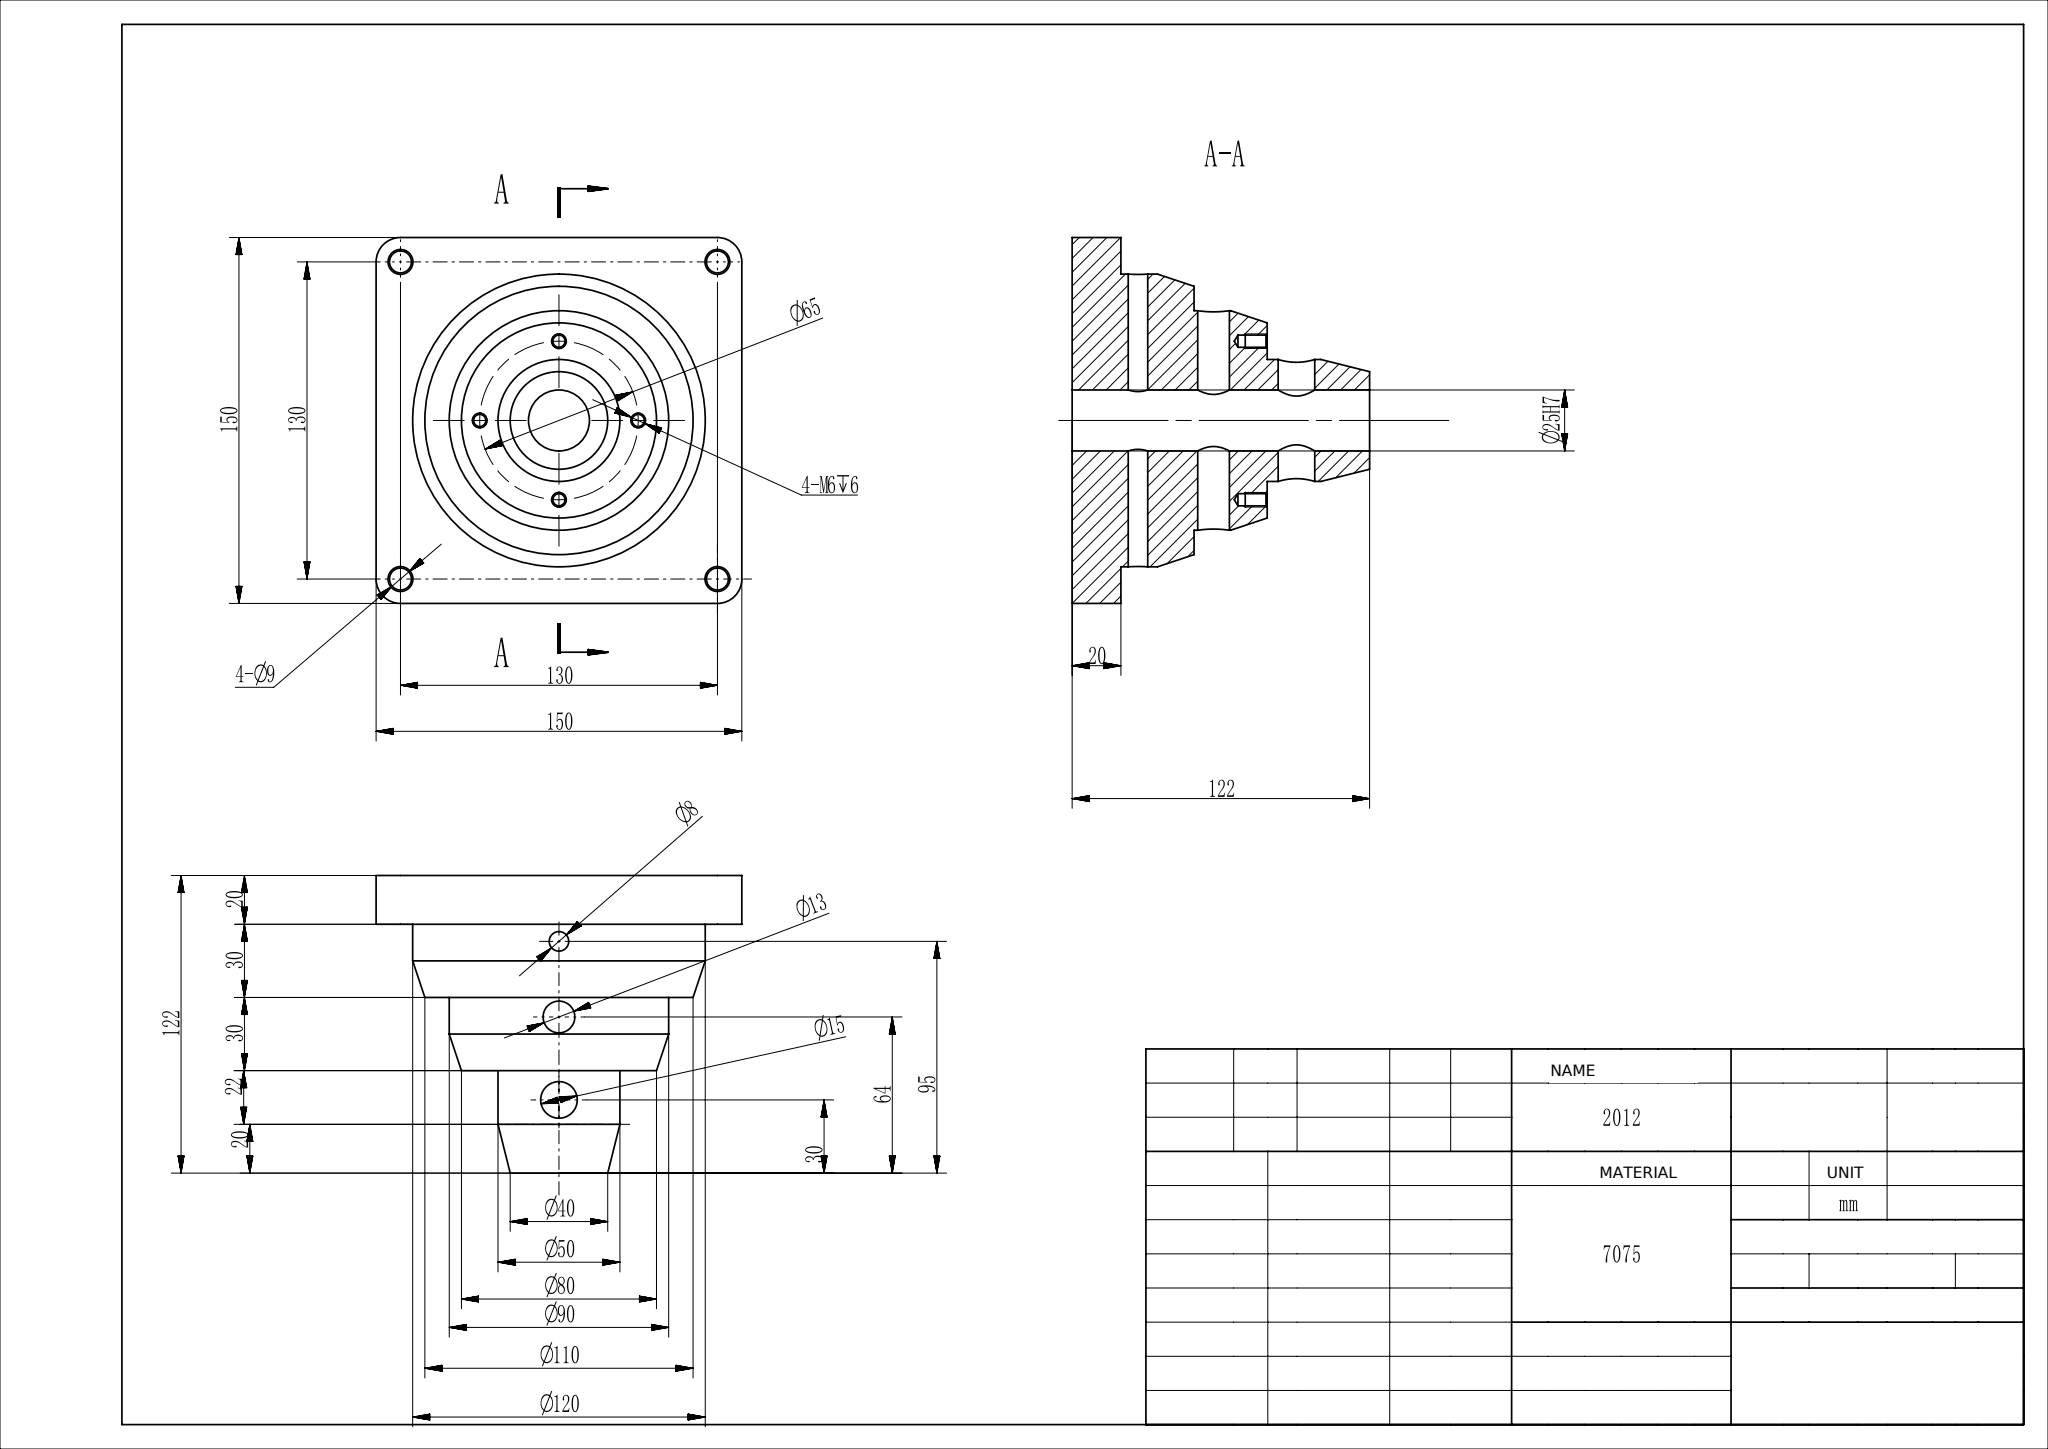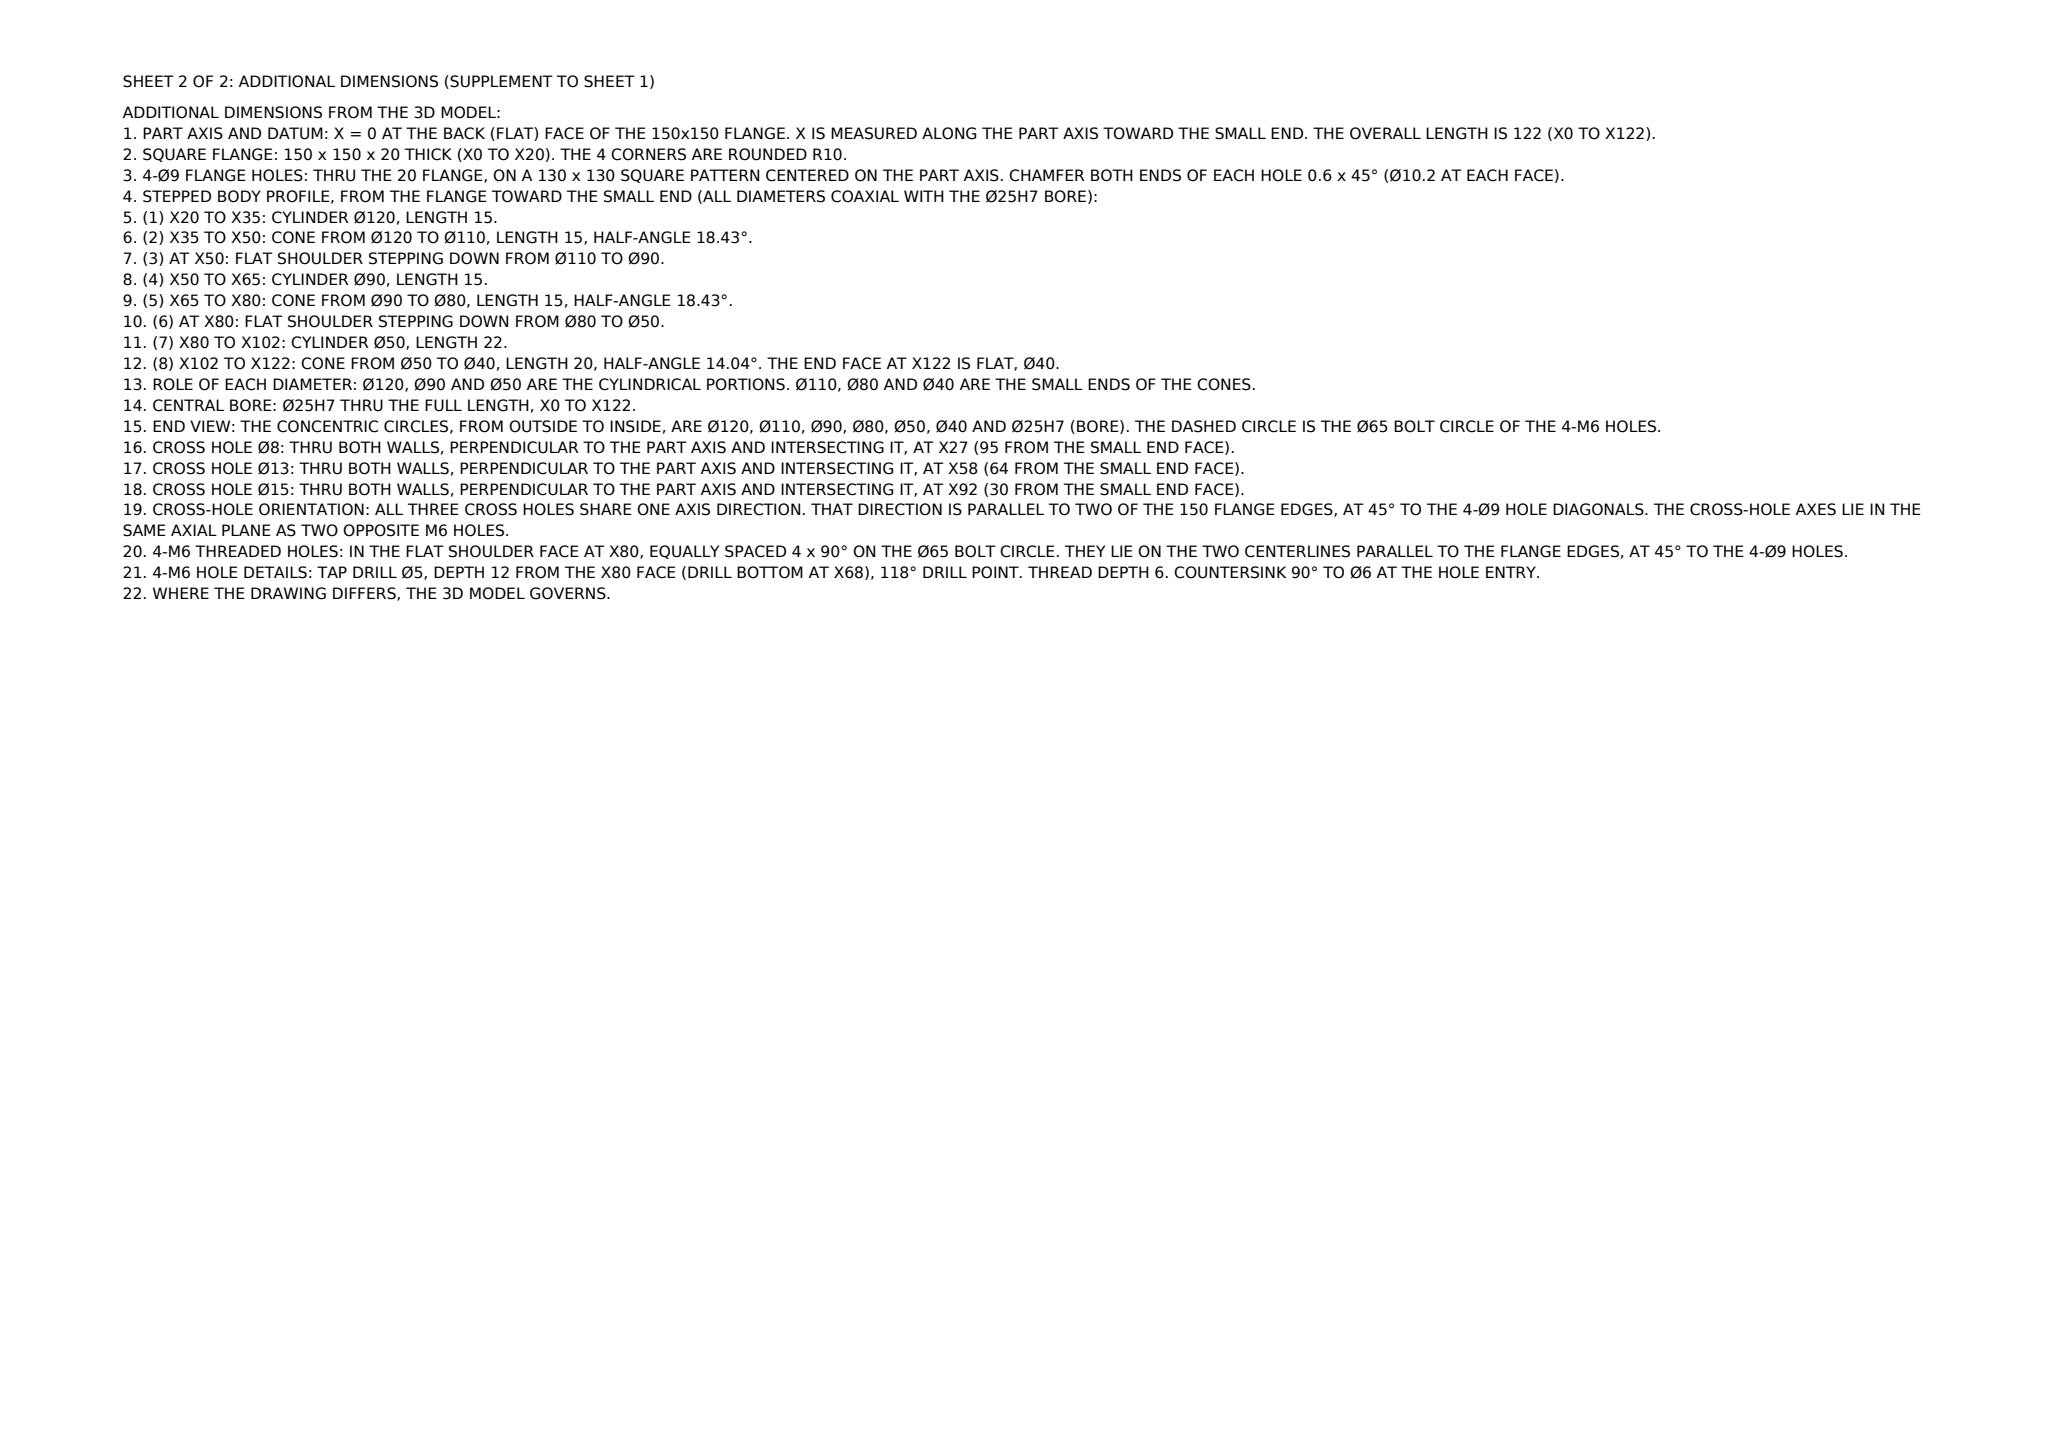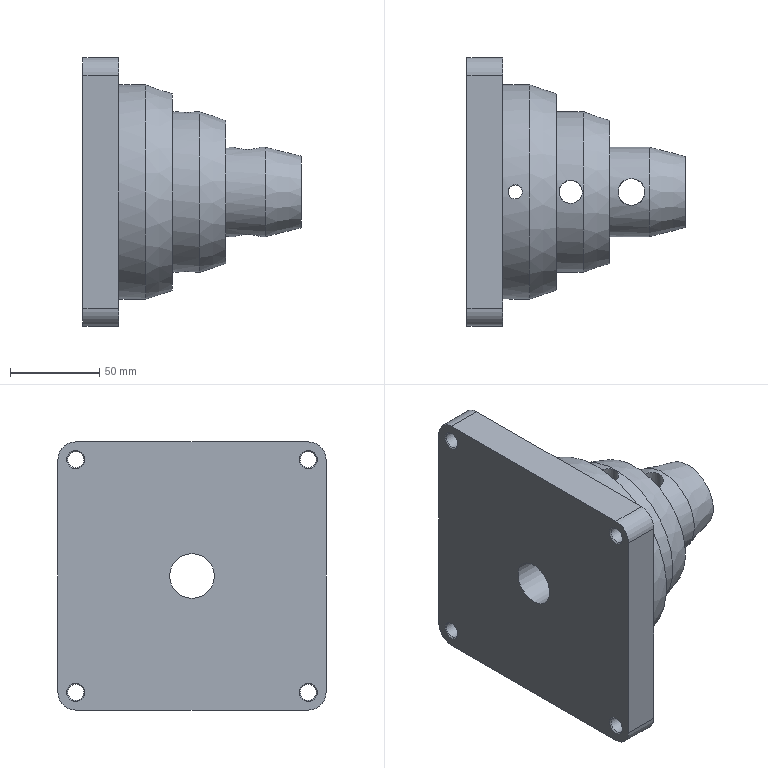Part | NX | mm | 1 solid | 50 faces | box 122 x 150 x 150 mm | volume 945575 mm3 | cylinder 22 | cone 19 | plane 9 | commonest cylinder face diameters 20 x4 9 x4 5 x4 8 x2 13 x2 15 x2 25 x1 50 x1